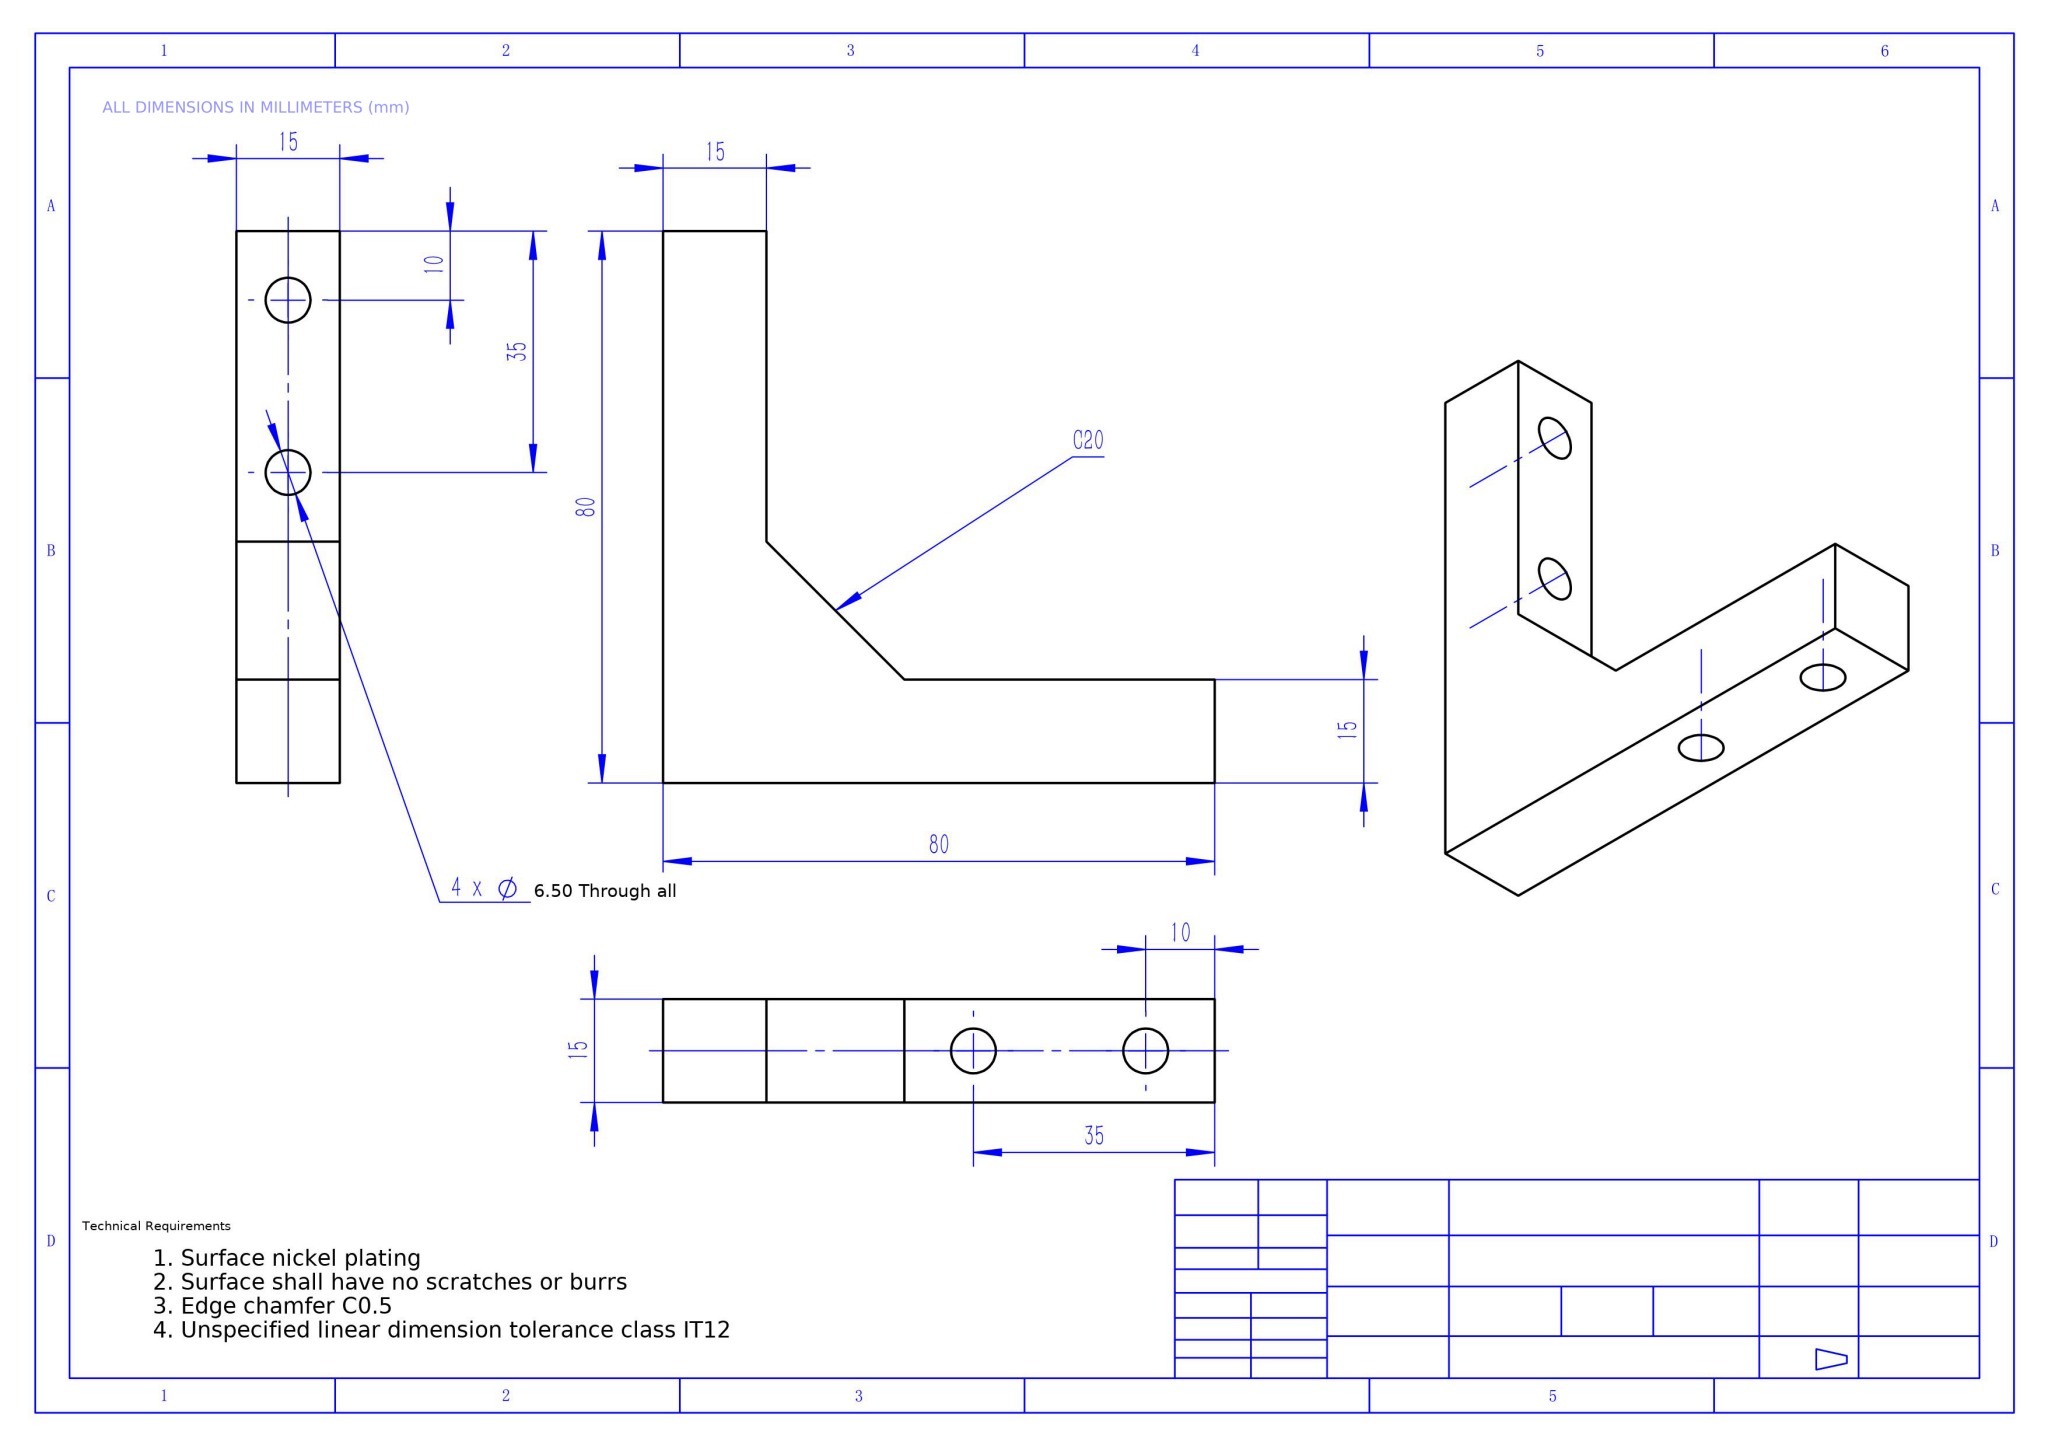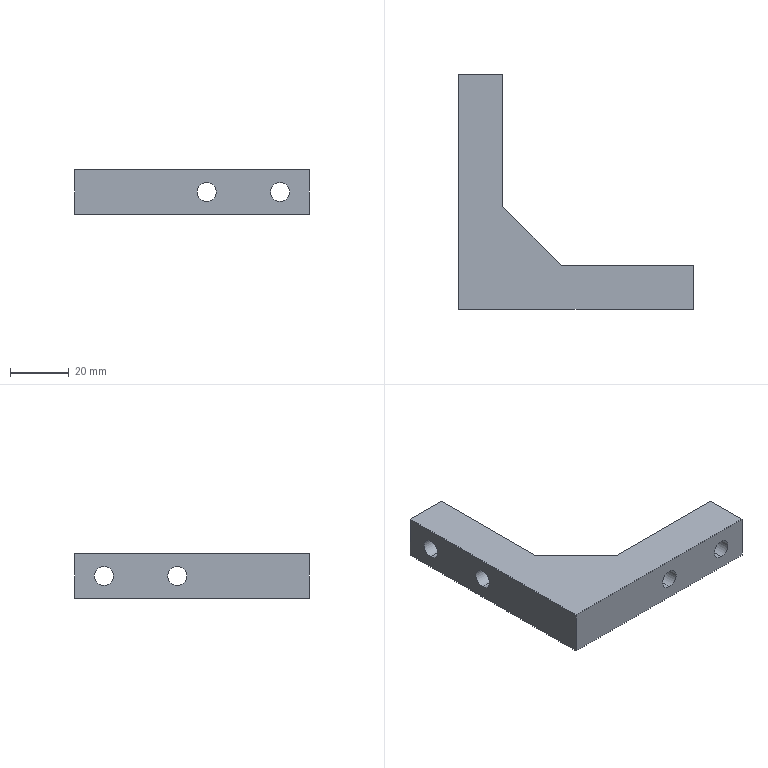Part | NX | mm | 1 solid | 17 faces | box 80 x 80 x 15 mm | volume 33634 mm3 | plane 9 | cylinder 8 | commonest cylinder face diameters 6.5 x8
STEP:
#1=COLOUR_RGB('',0.698,0.698,0.698);
#2=FILL_AREA_STYLE_COLOUR('',#1);
#3=FILL_AREA_STYLE('',(#2));
#4=SURFACE_STYLE_FILL_AREA(#3);
#5=SURFACE_SIDE_STYLE('',(#4));
#6=SURFACE_STYLE_USAGE(.BOTH.,#5);
#7=PRESENTATION_STYLE_ASSIGNMENT((#6));
#8=CARTESIAN_POINT('',(70.,0.,4.25));
#9=VERTEX_POINT('',#8);
#10=CARTESIAN_POINT('',(70.,0.,10.75));
#11=VERTEX_POINT('',#10);
#12=CARTESIAN_POINT('',(70.,0.,7.5));
#13=DIRECTION('',(0.,1.,0.));
#14=DIRECTION('',(0.,0.,1.));
#15=AXIS2_PLACEMENT_3D('',#12,#13,#14);
#16=CIRCLE('',#15,3.25);
#17=EDGE_CURVE('',#9,#11,#16,.T.);
#18=ORIENTED_EDGE('',*,*,#17,.F.);
#19=CARTESIAN_POINT('',(70.,15.,4.25));
#20=VERTEX_POINT('',#19);
#21=CARTESIAN_POINT('',(70.,15.,4.25));
#22=DIRECTION('',(0.,1.,0.));
#23=VECTOR('',#22,1000.);
#24=LINE('',#21,#23);
#25=EDGE_CURVE('',#9,#20,#24,.T.);
#26=ORIENTED_EDGE('',*,*,#25,.T.);
#27=CARTESIAN_POINT('',(70.,15.,10.75));
#28=VERTEX_POINT('',#27);
#29=CARTESIAN_POINT('',(70.,15.,7.5));
#30=DIRECTION('',(0.,1.,0.));
#31=DIRECTION('',(0.,0.,1.));
#32=AXIS2_PLACEMENT_3D('',#29,#30,#31);
#33=CIRCLE('',#32,3.25);
#34=EDGE_CURVE('',#20,#28,#33,.T.);
#35=ORIENTED_EDGE('',*,*,#34,.T.);
#36=CARTESIAN_POINT('',(70.,15.,10.75));
#37=DIRECTION('',(0.,1.,0.));
#38=VECTOR('',#37,1000.);
#39=LINE('',#36,#38);
#40=EDGE_CURVE('',#11,#28,#39,.T.);
#41=ORIENTED_EDGE('',*,*,#40,.F.);
#42=EDGE_LOOP('',(#18,#26,#35,#41));
#43=FACE_OUTER_BOUND('',#42,.T.);
#44=CARTESIAN_POINT('',(70.,15.,7.5));
#45=DIRECTION('',(0.,1.,0.));
#46=DIRECTION('',(0.,0.,1.));
#47=AXIS2_PLACEMENT_3D('',#44,#45,#46);
#48=CYLINDRICAL_SURFACE('',#47,3.25);
#49=ADVANCED_FACE('',(#43),#48,.F.);
#50=CARTESIAN_POINT('',(45.,0.,4.25));
#51=VERTEX_POINT('',#50);
#52=CARTESIAN_POINT('',(45.,0.,10.75));
#53=VERTEX_POINT('',#52);
#54=CARTESIAN_POINT('',(45.,0.,7.5));
#55=DIRECTION('',(0.,1.,0.));
#56=DIRECTION('',(0.,0.,1.));
#57=AXIS2_PLACEMENT_3D('',#54,#55,#56);
#58=CIRCLE('',#57,3.25);
#59=EDGE_CURVE('',#51,#53,#58,.T.);
#60=ORIENTED_EDGE('',*,*,#59,.F.);
#61=CARTESIAN_POINT('',(45.,15.,4.25));
#62=VERTEX_POINT('',#61);
#63=CARTESIAN_POINT('',(45.,15.,4.25));
#64=DIRECTION('',(0.,1.,0.));
#65=VECTOR('',#64,1000.);
#66=LINE('',#63,#65);
#67=EDGE_CURVE('',#51,#62,#66,.T.);
#68=ORIENTED_EDGE('',*,*,#67,.T.);
#69=CARTESIAN_POINT('',(45.,15.,10.75));
#70=VERTEX_POINT('',#69);
#71=CARTESIAN_POINT('',(45.,15.,7.5));
#72=DIRECTION('',(0.,1.,0.));
#73=DIRECTION('',(0.,0.,1.));
#74=AXIS2_PLACEMENT_3D('',#71,#72,#73);
#75=CIRCLE('',#74,3.25);
#76=EDGE_CURVE('',#62,#70,#75,.T.);
#77=ORIENTED_EDGE('',*,*,#76,.T.);
#78=CARTESIAN_POINT('',(45.,15.,10.75));
#79=DIRECTION('',(0.,1.,0.));
#80=VECTOR('',#79,1000.);
#81=LINE('',#78,#80);
#82=EDGE_CURVE('',#53,#70,#81,.T.);
#83=ORIENTED_EDGE('',*,*,#82,.F.);
#84=EDGE_LOOP('',(#60,#68,#77,#83));
#85=FACE_OUTER_BOUND('',#84,.T.);
#86=CARTESIAN_POINT('',(45.,15.,7.5));
#87=DIRECTION('',(0.,1.,0.));
#88=DIRECTION('',(0.,0.,1.));
#89=AXIS2_PLACEMENT_3D('',#86,#87,#88);
#90=CYLINDRICAL_SURFACE('',#89,3.25);
#91=ADVANCED_FACE('',(#85),#90,.F.);
#92=CARTESIAN_POINT('',(0.,45.,10.75));
#93=VERTEX_POINT('',#92);
#94=CARTESIAN_POINT('',(0.,45.,4.25));
#95=VERTEX_POINT('',#94);
#96=CARTESIAN_POINT('',(0.,45.,7.5));
#97=DIRECTION('',(1.,0.,0.));
#98=DIRECTION('',(0.,0.,-1.));
#99=AXIS2_PLACEMENT_3D('',#96,#97,#98);
#100=CIRCLE('',#99,3.25);
#101=EDGE_CURVE('',#93,#95,#100,.T.);
#102=ORIENTED_EDGE('',*,*,#101,.F.);
#103=CARTESIAN_POINT('',(15.,45.,10.75));
#104=VERTEX_POINT('',#103);
#105=CARTESIAN_POINT('',(15.,45.,10.75));
#106=DIRECTION('',(1.,0.,0.));
#107=VECTOR('',#106,1000.);
#108=LINE('',#105,#107);
#109=EDGE_CURVE('',#93,#104,#108,.T.);
#110=ORIENTED_EDGE('',*,*,#109,.T.);
#111=CARTESIAN_POINT('',(15.,45.,4.25));
#112=VERTEX_POINT('',#111);
#113=CARTESIAN_POINT('',(15.,45.,7.5));
#114=DIRECTION('',(1.,0.,0.));
#115=DIRECTION('',(0.,0.,-1.));
#116=AXIS2_PLACEMENT_3D('',#113,#114,#115);
#117=CIRCLE('',#116,3.25);
#118=EDGE_CURVE('',#104,#112,#117,.T.);
#119=ORIENTED_EDGE('',*,*,#118,.T.);
#120=CARTESIAN_POINT('',(15.,45.,4.25));
#121=DIRECTION('',(1.,0.,0.));
#122=VECTOR('',#121,1000.);
#123=LINE('',#120,#122);
#124=EDGE_CURVE('',#95,#112,#123,.T.);
#125=ORIENTED_EDGE('',*,*,#124,.F.);
#126=EDGE_LOOP('',(#102,#110,#119,#125));
#127=FACE_OUTER_BOUND('',#126,.T.);
#128=CARTESIAN_POINT('',(15.,45.,7.5));
#129=DIRECTION('',(1.,0.,0.));
#130=DIRECTION('',(0.,0.,-1.));
#131=AXIS2_PLACEMENT_3D('',#128,#129,#130);
#132=CYLINDRICAL_SURFACE('',#131,3.25);
#133=ADVANCED_FACE('',(#127),#132,.F.);
#134=CARTESIAN_POINT('',(0.,70.,10.75));
#135=VERTEX_POINT('',#134);
#136=CARTESIAN_POINT('',(0.,70.,4.25));
#137=VERTEX_POINT('',#136);
#138=CARTESIAN_POINT('',(0.,70.,7.5));
#139=DIRECTION('',(1.,0.,0.));
#140=DIRECTION('',(0.,0.,-1.));
#141=AXIS2_PLACEMENT_3D('',#138,#139,#140);
#142=CIRCLE('',#141,3.25);
#143=EDGE_CURVE('',#135,#137,#142,.T.);
#144=ORIENTED_EDGE('',*,*,#143,.F.);
#145=CARTESIAN_POINT('',(15.,70.,10.75));
#146=VERTEX_POINT('',#145);
#147=CARTESIAN_POINT('',(15.,70.,10.75));
#148=DIRECTION('',(1.,0.,0.));
#149=VECTOR('',#148,1000.);
#150=LINE('',#147,#149);
#151=EDGE_CURVE('',#135,#146,#150,.T.);
#152=ORIENTED_EDGE('',*,*,#151,.T.);
#153=CARTESIAN_POINT('',(15.,70.,4.25));
#154=VERTEX_POINT('',#153);
#155=CARTESIAN_POINT('',(15.,70.,7.5));
#156=DIRECTION('',(1.,0.,0.));
#157=DIRECTION('',(0.,0.,-1.));
#158=AXIS2_PLACEMENT_3D('',#155,#156,#157);
#159=CIRCLE('',#158,3.25);
#160=EDGE_CURVE('',#146,#154,#159,.T.);
#161=ORIENTED_EDGE('',*,*,#160,.T.);
#162=CARTESIAN_POINT('',(15.,70.,4.25));
#163=DIRECTION('',(1.,0.,0.));
#164=VECTOR('',#163,1000.);
#165=LINE('',#162,#164);
#166=EDGE_CURVE('',#137,#154,#165,.T.);
#167=ORIENTED_EDGE('',*,*,#166,.F.);
#168=EDGE_LOOP('',(#144,#152,#161,#167));
#169=FACE_OUTER_BOUND('',#168,.T.);
#170=CARTESIAN_POINT('',(15.,70.,7.5));
#171=DIRECTION('',(1.,0.,0.));
#172=DIRECTION('',(0.,0.,-1.));
#173=AXIS2_PLACEMENT_3D('',#170,#171,#172);
#174=CYLINDRICAL_SURFACE('',#173,3.25);
#175=ADVANCED_FACE('',(#169),#174,.F.);
#176=CARTESIAN_POINT('',(70.,0.,7.5));
#177=DIRECTION('',(0.,1.,0.));
#178=DIRECTION('',(0.,0.,1.));
#179=AXIS2_PLACEMENT_3D('',#176,#177,#178);
#180=CIRCLE('',#179,3.25);
#181=EDGE_CURVE('',#11,#9,#180,.T.);
#182=ORIENTED_EDGE('',*,*,#181,.T.);
#183=ORIENTED_EDGE('',*,*,#17,.T.);
#184=EDGE_LOOP('',(#182,#183));
#185=FACE_BOUND('',#184,.T.);
#186=CARTESIAN_POINT('',(45.,0.,7.5));
#187=DIRECTION('',(0.,1.,0.));
#188=DIRECTION('',(0.,0.,1.));
#189=AXIS2_PLACEMENT_3D('',#186,#187,#188);
#190=CIRCLE('',#189,3.25);
#191=EDGE_CURVE('',#53,#51,#190,.T.);
#192=ORIENTED_EDGE('',*,*,#191,.T.);
#193=ORIENTED_EDGE('',*,*,#59,.T.);
#194=EDGE_LOOP('',(#192,#193));
#195=FACE_BOUND('',#194,.T.);
#196=CARTESIAN_POINT('',(0.,0.,0.));
#197=VERTEX_POINT('',#196);
#198=CARTESIAN_POINT('',(80.,0.,0.));
#199=VERTEX_POINT('',#198);
#200=CARTESIAN_POINT('',(80.,0.,0.));
#201=DIRECTION('',(1.,0.,0.));
#202=VECTOR('',#201,1000.);
#203=LINE('',#200,#202);
#204=EDGE_CURVE('',#197,#199,#203,.T.);
#205=ORIENTED_EDGE('',*,*,#204,.T.);
#206=CARTESIAN_POINT('',(80.,0.,15.));
#207=VERTEX_POINT('',#206);
#208=CARTESIAN_POINT('',(80.,0.,15.));
#209=DIRECTION('',(0.,0.,-1.));
#210=VECTOR('',#209,1000.);
#211=LINE('',#208,#210);
#212=EDGE_CURVE('',#207,#199,#211,.T.);
#213=ORIENTED_EDGE('',*,*,#212,.F.);
#214=CARTESIAN_POINT('',(0.,0.,15.));
#215=VERTEX_POINT('',#214);
#216=CARTESIAN_POINT('',(80.,0.,15.));
#217=DIRECTION('',(1.,0.,0.));
#218=VECTOR('',#217,1000.);
#219=LINE('',#216,#218);
#220=EDGE_CURVE('',#215,#207,#219,.T.);
#221=ORIENTED_EDGE('',*,*,#220,.F.);
#222=CARTESIAN_POINT('',(0.,0.,15.));
#223=DIRECTION('',(0.,0.,-1.));
#224=VECTOR('',#223,1000.);
#225=LINE('',#222,#224);
#226=EDGE_CURVE('',#215,#197,#225,.T.);
#227=ORIENTED_EDGE('',*,*,#226,.T.);
#228=EDGE_LOOP('',(#205,#213,#221,#227));
#229=FACE_OUTER_BOUND('',#228,.T.);
#230=CARTESIAN_POINT('',(80.,0.,15.));
#231=DIRECTION('',(-0.,1.,0.));
#232=DIRECTION('',(-1.,-0.,0.));
#233=AXIS2_PLACEMENT_3D('',#230,#231,#232);
#234=PLANE('',#233);
#235=ADVANCED_FACE('',(#185,#195,#229),#234,.F.);
#236=CARTESIAN_POINT('',(80.,15.,0.));
#237=VERTEX_POINT('',#236);
#238=CARTESIAN_POINT('',(80.,15.,0.));
#239=DIRECTION('',(0.,1.,0.));
#240=VECTOR('',#239,1000.);
#241=LINE('',#238,#240);
#242=EDGE_CURVE('',#199,#237,#241,.T.);
#243=ORIENTED_EDGE('',*,*,#242,.T.);
#244=CARTESIAN_POINT('',(80.,15.,15.));
#245=VERTEX_POINT('',#244);
#246=CARTESIAN_POINT('',(80.,15.,15.));
#247=DIRECTION('',(0.,0.,-1.));
#248=VECTOR('',#247,1000.);
#249=LINE('',#246,#248);
#250=EDGE_CURVE('',#245,#237,#249,.T.);
#251=ORIENTED_EDGE('',*,*,#250,.F.);
#252=CARTESIAN_POINT('',(80.,15.,15.));
#253=DIRECTION('',(0.,1.,0.));
#254=VECTOR('',#253,1000.);
#255=LINE('',#252,#254);
#256=EDGE_CURVE('',#207,#245,#255,.T.);
#257=ORIENTED_EDGE('',*,*,#256,.F.);
#258=ORIENTED_EDGE('',*,*,#212,.T.);
#259=EDGE_LOOP('',(#243,#251,#257,#258));
#260=FACE_OUTER_BOUND('',#259,.T.);
#261=CARTESIAN_POINT('',(80.,15.,15.));
#262=DIRECTION('',(-1.,0.,0.));
#263=DIRECTION('',(0.,0.,1.));
#264=AXIS2_PLACEMENT_3D('',#261,#262,#263);
#265=PLANE('',#264);
#266=ADVANCED_FACE('',(#260),#265,.F.);
#267=CARTESIAN_POINT('',(70.,15.,7.5));
#268=DIRECTION('',(0.,1.,0.));
#269=DIRECTION('',(0.,0.,1.));
#270=AXIS2_PLACEMENT_3D('',#267,#268,#269);
#271=CIRCLE('',#270,3.25);
#272=EDGE_CURVE('',#28,#20,#271,.T.);
#273=ORIENTED_EDGE('',*,*,#272,.F.);
#274=ORIENTED_EDGE('',*,*,#34,.F.);
#275=EDGE_LOOP('',(#273,#274));
#276=FACE_BOUND('',#275,.T.);
#277=CARTESIAN_POINT('',(45.,15.,7.5));
#278=DIRECTION('',(0.,1.,0.));
#279=DIRECTION('',(0.,0.,1.));
#280=AXIS2_PLACEMENT_3D('',#277,#278,#279);
#281=CIRCLE('',#280,3.25);
#282=EDGE_CURVE('',#70,#62,#281,.T.);
#283=ORIENTED_EDGE('',*,*,#282,.F.);
#284=ORIENTED_EDGE('',*,*,#76,.F.);
#285=EDGE_LOOP('',(#283,#284));
#286=FACE_BOUND('',#285,.T.);
#287=CARTESIAN_POINT('',(35.,15.,0.));
#288=VERTEX_POINT('',#287);
#289=CARTESIAN_POINT('',(35.,15.,0.));
#290=DIRECTION('',(-1.,0.,0.));
#291=VECTOR('',#290,1000.);
#292=LINE('',#289,#291);
#293=EDGE_CURVE('',#237,#288,#292,.T.);
#294=ORIENTED_EDGE('',*,*,#293,.T.);
#295=CARTESIAN_POINT('',(35.,15.,15.));
#296=VERTEX_POINT('',#295);
#297=CARTESIAN_POINT('',(35.,15.,15.));
#298=DIRECTION('',(0.,0.,-1.));
#299=VECTOR('',#298,1000.);
#300=LINE('',#297,#299);
#301=EDGE_CURVE('',#296,#288,#300,.T.);
#302=ORIENTED_EDGE('',*,*,#301,.F.);
#303=CARTESIAN_POINT('',(35.,15.,15.));
#304=DIRECTION('',(-1.,0.,0.));
#305=VECTOR('',#304,1000.);
#306=LINE('',#303,#305);
#307=EDGE_CURVE('',#245,#296,#306,.T.);
#308=ORIENTED_EDGE('',*,*,#307,.F.);
#309=ORIENTED_EDGE('',*,*,#250,.T.);
#310=EDGE_LOOP('',(#294,#302,#308,#309));
#311=FACE_OUTER_BOUND('',#310,.T.);
#312=CARTESIAN_POINT('',(35.,15.,15.));
#313=DIRECTION('',(0.,-1.,0.));
#314=DIRECTION('',(0.,0.,-1.));
#315=AXIS2_PLACEMENT_3D('',#312,#313,#314);
#316=PLANE('',#315);
#317=ADVANCED_FACE('',(#276,#286,#311),#316,.F.);
#318=CARTESIAN_POINT('',(15.,35.,0.));
#319=VERTEX_POINT('',#318);
#320=CARTESIAN_POINT('',(15.,35.,0.));
#321=DIRECTION('',(-0.7071,0.7071,0.));
#322=VECTOR('',#321,1000.);
#323=LINE('',#320,#322);
#324=EDGE_CURVE('',#288,#319,#323,.T.);
#325=ORIENTED_EDGE('',*,*,#324,.T.);
#326=CARTESIAN_POINT('',(15.,35.,15.));
#327=VERTEX_POINT('',#326);
#328=CARTESIAN_POINT('',(15.,35.,15.));
#329=DIRECTION('',(0.,0.,-1.));
#330=VECTOR('',#329,1000.);
#331=LINE('',#328,#330);
#332=EDGE_CURVE('',#327,#319,#331,.T.);
#333=ORIENTED_EDGE('',*,*,#332,.F.);
#334=CARTESIAN_POINT('',(15.,35.,15.));
#335=DIRECTION('',(-0.7071,0.7071,0.));
#336=VECTOR('',#335,1000.);
#337=LINE('',#334,#336);
#338=EDGE_CURVE('',#296,#327,#337,.T.);
#339=ORIENTED_EDGE('',*,*,#338,.F.);
#340=ORIENTED_EDGE('',*,*,#301,.T.);
#341=EDGE_LOOP('',(#325,#333,#339,#340));
#342=FACE_OUTER_BOUND('',#341,.T.);
#343=CARTESIAN_POINT('',(15.,35.,15.));
#344=DIRECTION('',(-0.7071,-0.7071,0.));
#345=DIRECTION('',(0.7071,-0.7071,0.));
#346=AXIS2_PLACEMENT_3D('',#343,#344,#345);
#347=PLANE('',#346);
#348=ADVANCED_FACE('',(#342),#347,.F.);
#349=CARTESIAN_POINT('',(15.,45.,7.5));
#350=DIRECTION('',(1.,0.,0.));
#351=DIRECTION('',(0.,0.,-1.));
#352=AXIS2_PLACEMENT_3D('',#349,#350,#351);
#353=CIRCLE('',#352,3.25);
#354=EDGE_CURVE('',#112,#104,#353,.T.);
#355=ORIENTED_EDGE('',*,*,#354,.F.);
#356=ORIENTED_EDGE('',*,*,#118,.F.);
#357=EDGE_LOOP('',(#355,#356));
#358=FACE_BOUND('',#357,.T.);
#359=CARTESIAN_POINT('',(15.,70.,7.5));
#360=DIRECTION('',(1.,0.,0.));
#361=DIRECTION('',(0.,0.,-1.));
#362=AXIS2_PLACEMENT_3D('',#359,#360,#361);
#363=CIRCLE('',#362,3.25);
#364=EDGE_CURVE('',#154,#146,#363,.T.);
#365=ORIENTED_EDGE('',*,*,#364,.F.);
#366=ORIENTED_EDGE('',*,*,#160,.F.);
#367=EDGE_LOOP('',(#365,#366));
#368=FACE_BOUND('',#367,.T.);
#369=CARTESIAN_POINT('',(15.,80.,0.));
#370=VERTEX_POINT('',#369);
#371=CARTESIAN_POINT('',(15.,80.,0.));
#372=DIRECTION('',(-0.,1.,0.));
#373=VECTOR('',#372,1000.);
#374=LINE('',#371,#373);
#375=EDGE_CURVE('',#319,#370,#374,.T.);
#376=ORIENTED_EDGE('',*,*,#375,.T.);
#377=CARTESIAN_POINT('',(15.,80.,15.));
#378=VERTEX_POINT('',#377);
#379=CARTESIAN_POINT('',(15.,80.,15.));
#380=DIRECTION('',(0.,0.,-1.));
#381=VECTOR('',#380,1000.);
#382=LINE('',#379,#381);
#383=EDGE_CURVE('',#378,#370,#382,.T.);
#384=ORIENTED_EDGE('',*,*,#383,.F.);
#385=CARTESIAN_POINT('',(15.,80.,15.));
#386=DIRECTION('',(-0.,1.,0.));
#387=VECTOR('',#386,1000.);
#388=LINE('',#385,#387);
#389=EDGE_CURVE('',#327,#378,#388,.T.);
#390=ORIENTED_EDGE('',*,*,#389,.F.);
#391=ORIENTED_EDGE('',*,*,#332,.T.);
#392=EDGE_LOOP('',(#376,#384,#390,#391));
#393=FACE_OUTER_BOUND('',#392,.T.);
#394=CARTESIAN_POINT('',(15.,80.,15.));
#395=DIRECTION('',(-1.,-0.,0.));
#396=DIRECTION('',(0.,-1.,0.));
#397=AXIS2_PLACEMENT_3D('',#394,#395,#396);
#398=PLANE('',#397);
#399=ADVANCED_FACE('',(#358,#368,#393),#398,.F.);
#400=CARTESIAN_POINT('',(0.,80.,0.));
#401=VERTEX_POINT('',#400);
#402=CARTESIAN_POINT('',(0.,80.,0.));
#403=DIRECTION('',(-1.,0.,0.));
#404=VECTOR('',#403,1000.);
#405=LINE('',#402,#404);
#406=EDGE_CURVE('',#370,#401,#405,.T.);
#407=ORIENTED_EDGE('',*,*,#406,.T.);
#408=CARTESIAN_POINT('',(0.,80.,15.));
#409=VERTEX_POINT('',#408);
#410=CARTESIAN_POINT('',(0.,80.,15.));
#411=DIRECTION('',(0.,0.,-1.));
#412=VECTOR('',#411,1000.);
#413=LINE('',#410,#412);
#414=EDGE_CURVE('',#409,#401,#413,.T.);
#415=ORIENTED_EDGE('',*,*,#414,.F.);
#416=CARTESIAN_POINT('',(0.,80.,15.));
#417=DIRECTION('',(-1.,0.,0.));
#418=VECTOR('',#417,1000.);
#419=LINE('',#416,#418);
#420=EDGE_CURVE('',#378,#409,#419,.T.);
#421=ORIENTED_EDGE('',*,*,#420,.F.);
#422=ORIENTED_EDGE('',*,*,#383,.T.);
#423=EDGE_LOOP('',(#407,#415,#421,#422));
#424=FACE_OUTER_BOUND('',#423,.T.);
#425=CARTESIAN_POINT('',(0.,80.,15.));
#426=DIRECTION('',(0.,-1.,0.));
#427=DIRECTION('',(0.,0.,-1.));
#428=AXIS2_PLACEMENT_3D('',#425,#426,#427);
#429=PLANE('',#428);
#430=ADVANCED_FACE('',(#424),#429,.F.);
#431=CARTESIAN_POINT('',(0.,45.,7.5));
#432=DIRECTION('',(1.,0.,0.));
#433=DIRECTION('',(0.,0.,-1.));
#434=AXIS2_PLACEMENT_3D('',#431,#432,#433);
#435=CIRCLE('',#434,3.25);
#436=EDGE_CURVE('',#95,#93,#435,.T.);
#437=ORIENTED_EDGE('',*,*,#436,.T.);
#438=ORIENTED_EDGE('',*,*,#101,.T.);
#439=EDGE_LOOP('',(#437,#438));
#440=FACE_BOUND('',#439,.T.);
#441=CARTESIAN_POINT('',(0.,70.,7.5));
#442=DIRECTION('',(1.,0.,0.));
#443=DIRECTION('',(0.,0.,-1.));
#444=AXIS2_PLACEMENT_3D('',#441,#442,#443);
#445=CIRCLE('',#444,3.25);
#446=EDGE_CURVE('',#137,#135,#445,.T.);
#447=ORIENTED_EDGE('',*,*,#446,.T.);
#448=ORIENTED_EDGE('',*,*,#143,.T.);
#449=EDGE_LOOP('',(#447,#448));
#450=FACE_BOUND('',#449,.T.);
#451=CARTESIAN_POINT('',(0.,0.,0.));
#452=DIRECTION('',(0.,-1.,0.));
#453=VECTOR('',#452,1000.);
#454=LINE('',#451,#453);
#455=EDGE_CURVE('',#401,#197,#454,.T.);
#456=ORIENTED_EDGE('',*,*,#455,.T.);
#457=ORIENTED_EDGE('',*,*,#226,.F.);
#458=CARTESIAN_POINT('',(0.,0.,15.));
#459=DIRECTION('',(0.,-1.,0.));
#460=VECTOR('',#459,1000.);
#461=LINE('',#458,#460);
#462=EDGE_CURVE('',#409,#215,#461,.T.);
#463=ORIENTED_EDGE('',*,*,#462,.F.);
#464=ORIENTED_EDGE('',*,*,#414,.T.);
#465=EDGE_LOOP('',(#456,#457,#463,#464));
#466=FACE_OUTER_BOUND('',#465,.T.);
#467=CARTESIAN_POINT('',(0.,0.,15.));
#468=DIRECTION('',(1.,0.,0.));
#469=DIRECTION('',(0.,0.,-1.));
#470=AXIS2_PLACEMENT_3D('',#467,#468,#469);
#471=PLANE('',#470);
#472=ADVANCED_FACE('',(#440,#450,#466),#471,.F.);
#473=ORIENTED_EDGE('',*,*,#220,.T.);
#474=ORIENTED_EDGE('',*,*,#256,.T.);
#475=ORIENTED_EDGE('',*,*,#307,.T.);
#476=ORIENTED_EDGE('',*,*,#338,.T.);
#477=ORIENTED_EDGE('',*,*,#389,.T.);
#478=ORIENTED_EDGE('',*,*,#420,.T.);
#479=ORIENTED_EDGE('',*,*,#462,.T.);
#480=EDGE_LOOP('',(#473,#474,#475,#476,#477,#478,#479));
#481=FACE_OUTER_BOUND('',#480,.T.);
#482=CARTESIAN_POINT('',(0.,0.,15.));
#483=DIRECTION('',(0.,0.,-1.));
#484=DIRECTION('',(-1.,0.,0.));
#485=AXIS2_PLACEMENT_3D('',#482,#483,#484);
#486=PLANE('',#485);
#487=ADVANCED_FACE('',(#481),#486,.F.);
#488=ORIENTED_EDGE('',*,*,#204,.F.);
#489=ORIENTED_EDGE('',*,*,#455,.F.);
#490=ORIENTED_EDGE('',*,*,#406,.F.);
#491=ORIENTED_EDGE('',*,*,#375,.F.);
#492=ORIENTED_EDGE('',*,*,#324,.F.);
#493=ORIENTED_EDGE('',*,*,#293,.F.);
#494=ORIENTED_EDGE('',*,*,#242,.F.);
#495=EDGE_LOOP('',(#488,#489,#490,#491,#492,#493,#494));
#496=FACE_OUTER_BOUND('',#495,.T.);
#497=CARTESIAN_POINT('',(0.,0.,0.));
#498=DIRECTION('',(0.,0.,-1.));
#499=DIRECTION('',(-1.,0.,0.));
#500=AXIS2_PLACEMENT_3D('',#497,#498,#499);
#501=PLANE('',#500);
#502=ADVANCED_FACE('',(#496),#501,.T.);
#503=ORIENTED_EDGE('',*,*,#151,.F.);
#504=ORIENTED_EDGE('',*,*,#446,.F.);
#505=ORIENTED_EDGE('',*,*,#166,.T.);
#506=ORIENTED_EDGE('',*,*,#364,.T.);
#507=EDGE_LOOP('',(#503,#504,#505,#506));
#508=FACE_OUTER_BOUND('',#507,.T.);
#509=CARTESIAN_POINT('',(15.,70.,7.5));
#510=DIRECTION('',(1.,0.,0.));
#511=DIRECTION('',(0.,0.,-1.));
#512=AXIS2_PLACEMENT_3D('',#509,#510,#511);
#513=CYLINDRICAL_SURFACE('',#512,3.25);
#514=ADVANCED_FACE('',(#508),#513,.F.);
#515=ORIENTED_EDGE('',*,*,#109,.F.);
#516=ORIENTED_EDGE('',*,*,#436,.F.);
#517=ORIENTED_EDGE('',*,*,#124,.T.);
#518=ORIENTED_EDGE('',*,*,#354,.T.);
#519=EDGE_LOOP('',(#515,#516,#517,#518));
#520=FACE_OUTER_BOUND('',#519,.T.);
#521=CARTESIAN_POINT('',(15.,45.,7.5));
#522=DIRECTION('',(1.,0.,0.));
#523=DIRECTION('',(0.,0.,-1.));
#524=AXIS2_PLACEMENT_3D('',#521,#522,#523);
#525=CYLINDRICAL_SURFACE('',#524,3.25);
#526=ADVANCED_FACE('',(#520),#525,.F.);
#527=ORIENTED_EDGE('',*,*,#67,.F.);
#528=ORIENTED_EDGE('',*,*,#191,.F.);
#529=ORIENTED_EDGE('',*,*,#82,.T.);
#530=ORIENTED_EDGE('',*,*,#282,.T.);
#531=EDGE_LOOP('',(#527,#528,#529,#530));
#532=FACE_OUTER_BOUND('',#531,.T.);
#533=CARTESIAN_POINT('',(45.,15.,7.5));
#534=DIRECTION('',(0.,1.,0.));
#535=DIRECTION('',(0.,0.,1.));
#536=AXIS2_PLACEMENT_3D('',#533,#534,#535);
#537=CYLINDRICAL_SURFACE('',#536,3.25);
#538=ADVANCED_FACE('',(#532),#537,.F.);
#539=ORIENTED_EDGE('',*,*,#25,.F.);
#540=ORIENTED_EDGE('',*,*,#181,.F.);
#541=ORIENTED_EDGE('',*,*,#40,.T.);
#542=ORIENTED_EDGE('',*,*,#272,.T.);
#543=EDGE_LOOP('',(#539,#540,#541,#542));
#544=FACE_OUTER_BOUND('',#543,.T.);
#545=CARTESIAN_POINT('',(70.,15.,7.5));
#546=DIRECTION('',(0.,1.,0.));
#547=DIRECTION('',(0.,0.,1.));
#548=AXIS2_PLACEMENT_3D('',#545,#546,#547);
#549=CYLINDRICAL_SURFACE('',#548,3.25);
#550=ADVANCED_FACE('',(#544),#549,.F.);
#551=CLOSED_SHELL('',(#49,#91,#133,#175,#235,#266,#317,#348,#399,#430,#472,#487,#502,#514,#526,#538,#550));
#552=MANIFOLD_SOLID_BREP('',#551);
#553=CARTESIAN_POINT('',(0.,0.,0.));
#554=DIRECTION('',(0.,0.,1.));
#555=DIRECTION('',(1.,0.,0.));
#556=AXIS2_PLACEMENT_3D('',#553,#554,#555);
#557=(LENGTH_UNIT()NAMED_UNIT(*)SI_UNIT(.MILLI.,.METRE.));
#558=UNCERTAINTY_MEASURE_WITH_UNIT(LENGTH_MEASURE(0.00001),#557,'','');
#559=(NAMED_UNIT(*)PLANE_ANGLE_UNIT()SI_UNIT($,.RADIAN.));
#560=(NAMED_UNIT(*)SI_UNIT($,.STERADIAN.)SOLID_ANGLE_UNIT());
#561=(GEOMETRIC_REPRESENTATION_CONTEXT(3)GLOBAL_UNCERTAINTY_ASSIGNED_CONTEXT((#558))GLOBAL_UNIT_ASSIGNED_CONTEXT((#557,#559,#560))REPRESENTATION_CONTEXT('',''));
#562=ADVANCED_BREP_SHAPE_REPRESENTATION('',(#552,#556),#561);
#563=STYLED_ITEM('',(#7),#562);
#564=(LENGTH_UNIT()NAMED_UNIT(*)SI_UNIT(.MILLI.,.METRE.));
#565=UNCERTAINTY_MEASURE_WITH_UNIT(LENGTH_MEASURE(0.00001),#564,'','');
#566=(NAMED_UNIT(*)PLANE_ANGLE_UNIT()SI_UNIT($,.RADIAN.));
#567=(NAMED_UNIT(*)SI_UNIT($,.STERADIAN.)SOLID_ANGLE_UNIT());
#568=(GEOMETRIC_REPRESENTATION_CONTEXT(3)GLOBAL_UNCERTAINTY_ASSIGNED_CONTEXT((#565))GLOBAL_UNIT_ASSIGNED_CONTEXT((#564,#566,#567))REPRESENTATION_CONTEXT('',''));
#569=MECHANICAL_DESIGN_GEOMETRIC_PRESENTATION_REPRESENTATION('',(#563),#568);
#570=COLOUR_RGB('',0.698,0.698,0.698);
#571=FILL_AREA_STYLE_COLOUR('',#570);
#572=FILL_AREA_STYLE('',(#571));
#573=SURFACE_STYLE_FILL_AREA(#572);
#574=SURFACE_SIDE_STYLE('',(#573));
#575=SURFACE_STYLE_USAGE(.BOTH.,#574);
#576=PRESENTATION_STYLE_ASSIGNMENT((#575));
#577=STYLED_ITEM('',(#576),#552);
#578=PRESENTATION_LAYER_ASSIGNMENT('','',(#577));
#579=PRESENTATION_LAYER_ASSIGNMENT('','',(#563));
#580=(LENGTH_UNIT()NAMED_UNIT(*)SI_UNIT(.MILLI.,.METRE.));
#581=UNCERTAINTY_MEASURE_WITH_UNIT(LENGTH_MEASURE(0.00001),#580,'','');
#582=(NAMED_UNIT(*)PLANE_ANGLE_UNIT()SI_UNIT($,.RADIAN.));
#583=(NAMED_UNIT(*)SI_UNIT($,.STERADIAN.)SOLID_ANGLE_UNIT());
#584=(GEOMETRIC_REPRESENTATION_CONTEXT(3)GLOBAL_UNCERTAINTY_ASSIGNED_CONTEXT((#581))GLOBAL_UNIT_ASSIGNED_CONTEXT((#580,#582,#583))REPRESENTATION_CONTEXT('',''));
#585=MECHANICAL_DESIGN_GEOMETRIC_PRESENTATION_REPRESENTATION('',(#577),#584);